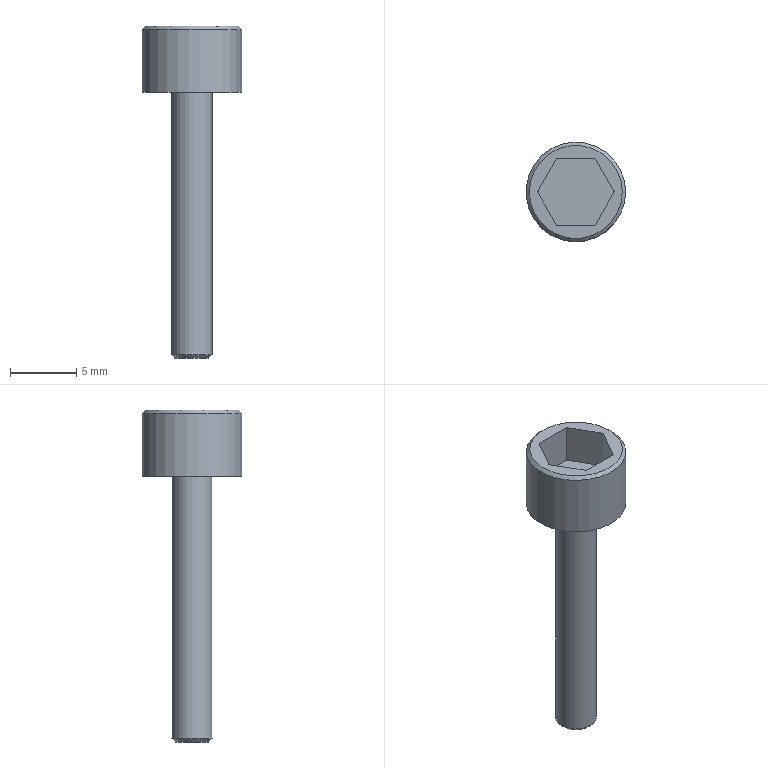Component | NX | SCREW | 1 solid | 14 faces | box 7.5 x 7.5 x 25 mm | volume 301 mm3 | plane 10 | cylinder 2 | cone 2 | commonest cylinder face diameters 3.045 x1 7.5 x1
STEP:
#1=CARTESIAN_POINT('',(0.,0.,0.));
#2=DIRECTION('',(0.,0.,1.));
#3=DIRECTION('',(1.,0.,0.));
#4=AXIS2_PLACEMENT_3D('',#1,#2,#3);
#5=CARTESIAN_POINT('',(23.5,-13.5,10.));
#6=VERTEX_POINT('',#5);
#7=CARTESIAN_POINT('',(20.,-13.5,10.));
#8=DIRECTION('',(0.,0.,1.));
#9=DIRECTION('',(1.,0.,0.));
#10=AXIS2_PLACEMENT_3D('',#7,#8,#9);
#11=CIRCLE('',#10,3.5);
#12=CARTESIAN_POINT('',(20.,-13.5,10.));
#13=DIRECTION('',(0.,0.,1.));
#14=DIRECTION('',(1.,0.,0.));
#15=AXIS2_PLACEMENT_3D('',#12,#13,#14);
#16=PLANE('',#15);
#17=CARTESIAN_POINT('',(0.,0.));
#18=DIRECTION('',(1.,0.));
#19=AXIS2_PLACEMENT_2D('',#17,#18);
#20=CIRCLE('',#19,3.5);
#21=(GEOMETRIC_REPRESENTATION_CONTEXT(2)PARAMETRIC_REPRESENTATION_CONTEXT()REPRESENTATION_CONTEXT('',''));
#22=DEFINITIONAL_REPRESENTATION('',(#20),#21);
#23=PCURVE('',#16,#22);
#24=CARTESIAN_POINT('',(20.,-13.5,10.));
#25=DIRECTION('',(0.,0.,-1.));
#26=DIRECTION('',(-1.,0.,0.));
#27=AXIS2_PLACEMENT_3D('',#24,#25,#26);
#28=CONICAL_SURFACE('',#27,3.5,0.7854);
#29=CARTESIAN_POINT('',(9.425,0.));
#30=DIRECTION('',(-1.,0.));
#31=VECTOR('',#30,1.);
#32=LINE('',#29,#31);
#33=(GEOMETRIC_REPRESENTATION_CONTEXT(2)PARAMETRIC_REPRESENTATION_CONTEXT()REPRESENTATION_CONTEXT('',''));
#34=DEFINITIONAL_REPRESENTATION('',(#32),#33);
#35=PCURVE('',#28,#34);
#36=SURFACE_CURVE('',#11,(#23,#35),.PCURVE_S1.);
#37=EDGE_CURVE('',#6,#6,#36,.T.);
#38=ORIENTED_EDGE('',*,*,#37,.T.);
#39=EDGE_LOOP('',(#38));
#40=FACE_BOUND('',#39,.T.);
#41=CARTESIAN_POINT('',(21.443,-11.,10.));
#42=VERTEX_POINT('',#41);
#43=CARTESIAN_POINT('',(22.887,-13.5,10.));
#44=VERTEX_POINT('',#43);
#45=CARTESIAN_POINT('',(21.443,-11.,10.));
#46=DIRECTION('',(0.5,-0.866,0.));
#47=VECTOR('',#46,1.);
#48=LINE('',#45,#47);
#49=CARTESIAN_POINT('',(1.443,2.5));
#50=DIRECTION('',(0.5,-0.866));
#51=VECTOR('',#50,1.);
#52=LINE('',#49,#51);
#53=(GEOMETRIC_REPRESENTATION_CONTEXT(2)PARAMETRIC_REPRESENTATION_CONTEXT()REPRESENTATION_CONTEXT('',''));
#54=DEFINITIONAL_REPRESENTATION('',(#52),#53);
#55=PCURVE('',#16,#54);
#56=CARTESIAN_POINT('',(21.443,-11.,7.));
#57=DIRECTION('',(-0.866,-0.5,0.));
#58=DIRECTION('',(0.5,-0.866,0.));
#59=AXIS2_PLACEMENT_3D('',#56,#57,#58);
#60=PLANE('',#59);
#61=CARTESIAN_POINT('',(0.,3.));
#62=DIRECTION('',(1.,0.));
#63=VECTOR('',#62,1.);
#64=LINE('',#61,#63);
#65=(GEOMETRIC_REPRESENTATION_CONTEXT(2)PARAMETRIC_REPRESENTATION_CONTEXT()REPRESENTATION_CONTEXT('',''));
#66=DEFINITIONAL_REPRESENTATION('',(#64),#65);
#67=PCURVE('',#60,#66);
#68=SURFACE_CURVE('',#48,(#55,#67),.PCURVE_S1.);
#69=EDGE_CURVE('',#42,#44,#68,.T.);
#70=ORIENTED_EDGE('',*,*,#69,.T.);
#71=CARTESIAN_POINT('',(21.443,-16.,10.));
#72=VERTEX_POINT('',#71);
#73=CARTESIAN_POINT('',(22.887,-13.5,10.));
#74=DIRECTION('',(-0.5,-0.866,0.));
#75=VECTOR('',#74,1.);
#76=LINE('',#73,#75);
#77=CARTESIAN_POINT('',(2.887,0.));
#78=DIRECTION('',(-0.5,-0.866));
#79=VECTOR('',#78,1.);
#80=LINE('',#77,#79);
#81=(GEOMETRIC_REPRESENTATION_CONTEXT(2)PARAMETRIC_REPRESENTATION_CONTEXT()REPRESENTATION_CONTEXT('',''));
#82=DEFINITIONAL_REPRESENTATION('',(#80),#81);
#83=PCURVE('',#16,#82);
#84=CARTESIAN_POINT('',(22.887,-13.5,7.));
#85=DIRECTION('',(-0.866,0.5,0.));
#86=DIRECTION('',(-0.5,-0.866,0.));
#87=AXIS2_PLACEMENT_3D('',#84,#85,#86);
#88=PLANE('',#87);
#89=CARTESIAN_POINT('',(0.,3.));
#90=DIRECTION('',(1.,0.));
#91=VECTOR('',#90,1.);
#92=LINE('',#89,#91);
#93=(GEOMETRIC_REPRESENTATION_CONTEXT(2)PARAMETRIC_REPRESENTATION_CONTEXT()REPRESENTATION_CONTEXT('',''));
#94=DEFINITIONAL_REPRESENTATION('',(#92),#93);
#95=PCURVE('',#88,#94);
#96=SURFACE_CURVE('',#76,(#83,#95),.PCURVE_S1.);
#97=EDGE_CURVE('',#44,#72,#96,.T.);
#98=ORIENTED_EDGE('',*,*,#97,.T.);
#99=CARTESIAN_POINT('',(18.557,-16.,10.));
#100=VERTEX_POINT('',#99);
#101=CARTESIAN_POINT('',(21.443,-16.,10.));
#102=DIRECTION('',(-1.,0.,0.));
#103=VECTOR('',#102,1.);
#104=LINE('',#101,#103);
#105=CARTESIAN_POINT('',(1.443,-2.5));
#106=DIRECTION('',(-1.,0.));
#107=VECTOR('',#106,1.);
#108=LINE('',#105,#107);
#109=(GEOMETRIC_REPRESENTATION_CONTEXT(2)PARAMETRIC_REPRESENTATION_CONTEXT()REPRESENTATION_CONTEXT('',''));
#110=DEFINITIONAL_REPRESENTATION('',(#108),#109);
#111=PCURVE('',#16,#110);
#112=CARTESIAN_POINT('',(21.443,-16.,7.));
#113=DIRECTION('',(0.,1.,0.));
#114=DIRECTION('',(-1.,0.,0.));
#115=AXIS2_PLACEMENT_3D('',#112,#113,#114);
#116=PLANE('',#115);
#117=CARTESIAN_POINT('',(0.,3.));
#118=DIRECTION('',(1.,0.));
#119=VECTOR('',#118,1.);
#120=LINE('',#117,#119);
#121=(GEOMETRIC_REPRESENTATION_CONTEXT(2)PARAMETRIC_REPRESENTATION_CONTEXT()REPRESENTATION_CONTEXT('',''));
#122=DEFINITIONAL_REPRESENTATION('',(#120),#121);
#123=PCURVE('',#116,#122);
#124=SURFACE_CURVE('',#104,(#111,#123),.PCURVE_S1.);
#125=EDGE_CURVE('',#72,#100,#124,.T.);
#126=ORIENTED_EDGE('',*,*,#125,.T.);
#127=CARTESIAN_POINT('',(17.113,-13.5,10.));
#128=VERTEX_POINT('',#127);
#129=CARTESIAN_POINT('',(18.557,-16.,10.));
#130=DIRECTION('',(-0.5,0.866,0.));
#131=VECTOR('',#130,1.);
#132=LINE('',#129,#131);
#133=CARTESIAN_POINT('',(-1.443,-2.5));
#134=DIRECTION('',(-0.5,0.866));
#135=VECTOR('',#134,1.);
#136=LINE('',#133,#135);
#137=(GEOMETRIC_REPRESENTATION_CONTEXT(2)PARAMETRIC_REPRESENTATION_CONTEXT()REPRESENTATION_CONTEXT('',''));
#138=DEFINITIONAL_REPRESENTATION('',(#136),#137);
#139=PCURVE('',#16,#138);
#140=CARTESIAN_POINT('',(18.557,-16.,7.));
#141=DIRECTION('',(0.866,0.5,0.));
#142=DIRECTION('',(-0.5,0.866,0.));
#143=AXIS2_PLACEMENT_3D('',#140,#141,#142);
#144=PLANE('',#143);
#145=CARTESIAN_POINT('',(0.,3.));
#146=DIRECTION('',(1.,0.));
#147=VECTOR('',#146,1.);
#148=LINE('',#145,#147);
#149=(GEOMETRIC_REPRESENTATION_CONTEXT(2)PARAMETRIC_REPRESENTATION_CONTEXT()REPRESENTATION_CONTEXT('',''));
#150=DEFINITIONAL_REPRESENTATION('',(#148),#149);
#151=PCURVE('',#144,#150);
#152=SURFACE_CURVE('',#132,(#139,#151),.PCURVE_S1.);
#153=EDGE_CURVE('',#100,#128,#152,.T.);
#154=ORIENTED_EDGE('',*,*,#153,.T.);
#155=CARTESIAN_POINT('',(18.557,-11.,10.));
#156=VERTEX_POINT('',#155);
#157=CARTESIAN_POINT('',(17.113,-13.5,10.));
#158=DIRECTION('',(0.5,0.866,0.));
#159=VECTOR('',#158,1.);
#160=LINE('',#157,#159);
#161=CARTESIAN_POINT('',(-2.887,0.));
#162=DIRECTION('',(0.5,0.866));
#163=VECTOR('',#162,1.);
#164=LINE('',#161,#163);
#165=(GEOMETRIC_REPRESENTATION_CONTEXT(2)PARAMETRIC_REPRESENTATION_CONTEXT()REPRESENTATION_CONTEXT('',''));
#166=DEFINITIONAL_REPRESENTATION('',(#164),#165);
#167=PCURVE('',#16,#166);
#168=CARTESIAN_POINT('',(17.113,-13.5,7.));
#169=DIRECTION('',(0.866,-0.5,0.));
#170=DIRECTION('',(0.5,0.866,0.));
#171=AXIS2_PLACEMENT_3D('',#168,#169,#170);
#172=PLANE('',#171);
#173=CARTESIAN_POINT('',(0.,3.));
#174=DIRECTION('',(1.,0.));
#175=VECTOR('',#174,1.);
#176=LINE('',#173,#175);
#177=(GEOMETRIC_REPRESENTATION_CONTEXT(2)PARAMETRIC_REPRESENTATION_CONTEXT()REPRESENTATION_CONTEXT('',''));
#178=DEFINITIONAL_REPRESENTATION('',(#176),#177);
#179=PCURVE('',#172,#178);
#180=SURFACE_CURVE('',#160,(#167,#179),.PCURVE_S1.);
#181=EDGE_CURVE('',#128,#156,#180,.T.);
#182=ORIENTED_EDGE('',*,*,#181,.T.);
#183=CARTESIAN_POINT('',(18.557,-11.,10.));
#184=DIRECTION('',(1.,0.,0.));
#185=VECTOR('',#184,1.);
#186=LINE('',#183,#185);
#187=CARTESIAN_POINT('',(-1.443,2.5));
#188=DIRECTION('',(1.,0.));
#189=VECTOR('',#188,1.);
#190=LINE('',#187,#189);
#191=(GEOMETRIC_REPRESENTATION_CONTEXT(2)PARAMETRIC_REPRESENTATION_CONTEXT()REPRESENTATION_CONTEXT('',''));
#192=DEFINITIONAL_REPRESENTATION('',(#190),#191);
#193=PCURVE('',#16,#192);
#194=CARTESIAN_POINT('',(18.557,-11.,7.));
#195=DIRECTION('',(0.,-1.,0.));
#196=DIRECTION('',(1.,0.,0.));
#197=AXIS2_PLACEMENT_3D('',#194,#195,#196);
#198=PLANE('',#197);
#199=CARTESIAN_POINT('',(0.,3.));
#200=DIRECTION('',(1.,0.));
#201=VECTOR('',#200,1.);
#202=LINE('',#199,#201);
#203=(GEOMETRIC_REPRESENTATION_CONTEXT(2)PARAMETRIC_REPRESENTATION_CONTEXT()REPRESENTATION_CONTEXT('',''));
#204=DEFINITIONAL_REPRESENTATION('',(#202),#203);
#205=PCURVE('',#198,#204);
#206=SURFACE_CURVE('',#186,(#193,#205),.PCURVE_S1.);
#207=EDGE_CURVE('',#156,#42,#206,.T.);
#208=ORIENTED_EDGE('',*,*,#207,.T.);
#209=EDGE_LOOP('',(#70,#98,#126,#154,#182,#208));
#210=FACE_BOUND('',#209,.T.);
#211=ADVANCED_FACE('',(#40,#210),#16,.T.);
#212=CARTESIAN_POINT('',(18.727,-13.5,-15.));
#213=VERTEX_POINT('',#212);
#214=CARTESIAN_POINT('',(20.,-13.5,-15.));
#215=DIRECTION('',(0.,0.,-1.));
#216=DIRECTION('',(-1.,0.,0.));
#217=AXIS2_PLACEMENT_3D('',#214,#215,#216);
#218=CIRCLE('',#217,1.273);
#219=CARTESIAN_POINT('',(20.,-13.5,-15.));
#220=DIRECTION('',(0.,0.,-1.));
#221=DIRECTION('',(-1.,0.,0.));
#222=AXIS2_PLACEMENT_3D('',#219,#220,#221);
#223=PLANE('',#222);
#224=CARTESIAN_POINT('',(0.,0.));
#225=DIRECTION('',(1.,0.));
#226=AXIS2_PLACEMENT_2D('',#224,#225);
#227=CIRCLE('',#226,1.273);
#228=(GEOMETRIC_REPRESENTATION_CONTEXT(2)PARAMETRIC_REPRESENTATION_CONTEXT()REPRESENTATION_CONTEXT('',''));
#229=DEFINITIONAL_REPRESENTATION('',(#227),#228);
#230=PCURVE('',#223,#229);
#231=CARTESIAN_POINT('',(20.,-13.5,-14.75));
#232=DIRECTION('',(0.,0.,1.));
#233=DIRECTION('',(1.,0.,0.));
#234=AXIS2_PLACEMENT_3D('',#231,#232,#233);
#235=CONICAL_SURFACE('',#234,1.523,0.7854);
#236=CARTESIAN_POINT('',(9.425,-0.25));
#237=DIRECTION('',(-1.,0.));
#238=VECTOR('',#237,1.);
#239=LINE('',#236,#238);
#240=(GEOMETRIC_REPRESENTATION_CONTEXT(2)PARAMETRIC_REPRESENTATION_CONTEXT()REPRESENTATION_CONTEXT('',''));
#241=DEFINITIONAL_REPRESENTATION('',(#239),#240);
#242=PCURVE('',#235,#241);
#243=SURFACE_CURVE('',#218,(#230,#242),.PCURVE_S1.);
#244=EDGE_CURVE('',#213,#213,#243,.T.);
#245=ORIENTED_EDGE('',*,*,#244,.T.);
#246=EDGE_LOOP('',(#245));
#247=FACE_BOUND('',#246,.T.);
#248=ADVANCED_FACE('',(#247),#223,.T.);
#249=CARTESIAN_POINT('',(18.477,-13.5,-14.75));
#250=VERTEX_POINT('',#249);
#251=CARTESIAN_POINT('',(21.523,-13.5,-14.75));
#252=VERTEX_POINT('',#251);
#253=CARTESIAN_POINT('',(20.,-13.5,-14.75));
#254=DIRECTION('',(0.,0.,1.));
#255=DIRECTION('',(-1.,0.,0.));
#256=AXIS2_PLACEMENT_3D('',#253,#254,#255);
#257=CIRCLE('',#256,1.523);
#258=CARTESIAN_POINT('',(20.,-13.5,-15.));
#259=DIRECTION('',(0.,0.,1.));
#260=DIRECTION('',(1.,0.,0.));
#261=AXIS2_PLACEMENT_3D('',#258,#259,#260);
#262=CYLINDRICAL_SURFACE('',#261,1.523);
#263=CARTESIAN_POINT('',(3.142,0.25));
#264=DIRECTION('',(1.,0.));
#265=VECTOR('',#264,1.);
#266=LINE('',#263,#265);
#267=(GEOMETRIC_REPRESENTATION_CONTEXT(2)PARAMETRIC_REPRESENTATION_CONTEXT()REPRESENTATION_CONTEXT('',''));
#268=DEFINITIONAL_REPRESENTATION('',(#266),#267);
#269=PCURVE('',#262,#268);
#270=CARTESIAN_POINT('',(3.142,-0.));
#271=DIRECTION('',(1.,0.));
#272=VECTOR('',#271,1.);
#273=LINE('',#270,#272);
#274=(GEOMETRIC_REPRESENTATION_CONTEXT(2)PARAMETRIC_REPRESENTATION_CONTEXT()REPRESENTATION_CONTEXT('',''));
#275=DEFINITIONAL_REPRESENTATION('',(#273),#274);
#276=PCURVE('',#235,#275);
#277=SURFACE_CURVE('',#257,(#269,#276),.PCURVE_S1.);
#278=EDGE_CURVE('',#250,#252,#277,.T.);
#279=ORIENTED_EDGE('',*,*,#278,.T.);
#280=CARTESIAN_POINT('',(21.523,-13.5,5.));
#281=VERTEX_POINT('',#280);
#282=CARTESIAN_POINT('',(21.523,-13.5,-14.75));
#283=CARTESIAN_POINT('',(21.523,-13.5,5.));
#284=B_SPLINE_CURVE_WITH_KNOTS('',1,(#282,#283),.UNSPECIFIED.,.F.,.F.,(2,2),(0.25,20.),.PIECEWISE_BEZIER_KNOTS.);
#285=CARTESIAN_POINT('',(6.283,0.));
#286=DIRECTION('',(0.,1.));
#287=VECTOR('',#286,1.);
#288=LINE('',#285,#287);
#289=(GEOMETRIC_REPRESENTATION_CONTEXT(2)PARAMETRIC_REPRESENTATION_CONTEXT()REPRESENTATION_CONTEXT('',''));
#290=DEFINITIONAL_REPRESENTATION('',(#288),#289);
#291=PCURVE('',#262,#290);
#292=CARTESIAN_POINT('',(0.,0.));
#293=DIRECTION('',(0.,1.));
#294=VECTOR('',#293,1.);
#295=LINE('',#292,#294);
#296=(GEOMETRIC_REPRESENTATION_CONTEXT(2)PARAMETRIC_REPRESENTATION_CONTEXT()REPRESENTATION_CONTEXT('',''));
#297=DEFINITIONAL_REPRESENTATION('',(#295),#296);
#298=PCURVE('',#262,#297);
#299=SEAM_CURVE('',#284,(#291,#298),.PCURVE_S1.);
#300=EDGE_CURVE('',#252,#281,#299,.T.);
#301=ORIENTED_EDGE('',*,*,#300,.T.);
#302=CARTESIAN_POINT('',(20.,-13.5,5.));
#303=DIRECTION('',(0.,0.,-1.));
#304=DIRECTION('',(1.,0.,0.));
#305=AXIS2_PLACEMENT_3D('',#302,#303,#304);
#306=CIRCLE('',#305,1.523);
#307=CARTESIAN_POINT('',(6.283,20.));
#308=DIRECTION('',(-1.,0.));
#309=VECTOR('',#308,1.);
#310=LINE('',#307,#309);
#311=(GEOMETRIC_REPRESENTATION_CONTEXT(2)PARAMETRIC_REPRESENTATION_CONTEXT()REPRESENTATION_CONTEXT('',''));
#312=DEFINITIONAL_REPRESENTATION('',(#310),#311);
#313=PCURVE('',#262,#312);
#314=CARTESIAN_POINT('',(20.,-13.5,5.));
#315=DIRECTION('',(0.,0.,-1.));
#316=DIRECTION('',(-1.,0.,0.));
#317=AXIS2_PLACEMENT_3D('',#314,#315,#316);
#318=PLANE('',#317);
#319=CARTESIAN_POINT('',(0.,0.));
#320=DIRECTION('',(-1.,0.));
#321=AXIS2_PLACEMENT_2D('',#319,#320);
#322=CIRCLE('',#321,1.523);
#323=(GEOMETRIC_REPRESENTATION_CONTEXT(2)PARAMETRIC_REPRESENTATION_CONTEXT()REPRESENTATION_CONTEXT('',''));
#324=DEFINITIONAL_REPRESENTATION('',(#322),#323);
#325=PCURVE('',#318,#324);
#326=SURFACE_CURVE('',#306,(#313,#325),.PCURVE_S1.);
#327=EDGE_CURVE('',#281,#281,#326,.T.);
#328=ORIENTED_EDGE('',*,*,#327,.T.);
#329=ORIENTED_EDGE('',*,*,#300,.F.);
#330=CARTESIAN_POINT('',(20.,-13.5,-14.75));
#331=DIRECTION('',(0.,0.,1.));
#332=DIRECTION('',(-1.,0.,0.));
#333=AXIS2_PLACEMENT_3D('',#330,#331,#332);
#334=CIRCLE('',#333,1.523);
#335=CARTESIAN_POINT('',(-3.142,0.25));
#336=DIRECTION('',(1.,0.));
#337=VECTOR('',#336,1.);
#338=LINE('',#335,#337);
#339=(GEOMETRIC_REPRESENTATION_CONTEXT(2)PARAMETRIC_REPRESENTATION_CONTEXT()REPRESENTATION_CONTEXT('',''));
#340=DEFINITIONAL_REPRESENTATION('',(#338),#339);
#341=PCURVE('',#262,#340);
#342=CARTESIAN_POINT('',(3.142,-0.));
#343=DIRECTION('',(1.,0.));
#344=VECTOR('',#343,1.);
#345=LINE('',#342,#344);
#346=(GEOMETRIC_REPRESENTATION_CONTEXT(2)PARAMETRIC_REPRESENTATION_CONTEXT()REPRESENTATION_CONTEXT('',''));
#347=DEFINITIONAL_REPRESENTATION('',(#345),#346);
#348=PCURVE('',#235,#347);
#349=SURFACE_CURVE('',#334,(#341,#348),.PCURVE_S1.);
#350=EDGE_CURVE('',#252,#250,#349,.T.);
#351=ORIENTED_EDGE('',*,*,#350,.T.);
#352=EDGE_LOOP('',(#279,#301,#328,#329,#351));
#353=FACE_BOUND('',#352,.T.);
#354=ADVANCED_FACE('',(#353),#262,.T.);
#355=ORIENTED_EDGE('',*,*,#327,.F.);
#356=EDGE_LOOP('',(#355));
#357=FACE_BOUND('',#356,.T.);
#358=CARTESIAN_POINT('',(23.75,-13.5,5.));
#359=VERTEX_POINT('',#358);
#360=CARTESIAN_POINT('',(20.,-13.5,5.));
#361=DIRECTION('',(0.,0.,1.));
#362=DIRECTION('',(1.,0.,0.));
#363=AXIS2_PLACEMENT_3D('',#360,#361,#362);
#364=CIRCLE('',#363,3.75);
#365=CARTESIAN_POINT('',(-3.75,0.));
#366=CARTESIAN_POINT('',(-3.75,6.495));
#367=CARTESIAN_POINT('',(1.875,3.248));
#368=CARTESIAN_POINT('',(7.5,0.));
#369=CARTESIAN_POINT('',(1.875,-3.248));
#370=CARTESIAN_POINT('',(-3.75,-6.495));
#371=CARTESIAN_POINT('',(-3.75,0.));
#372=(BOUNDED_CURVE()B_SPLINE_CURVE(2,(#365,#366,#367,#368,#369,#370,#371),.UNSPECIFIED.,.T.,.F.)B_SPLINE_CURVE_WITH_KNOTS((1,2,2,2,2,1),(-2.094,0.,2.094,4.189,6.283,8.378),.UNSPECIFIED.)CURVE()GEOMETRIC_REPRESENTATION_ITEM()RATIONAL_B_SPLINE_CURVE((1.,0.5,1.,0.5,1.,0.5,1.))REPRESENTATION_ITEM(''));
#373=(GEOMETRIC_REPRESENTATION_CONTEXT(2)PARAMETRIC_REPRESENTATION_CONTEXT()REPRESENTATION_CONTEXT('',''));
#374=DEFINITIONAL_REPRESENTATION('',(#372),#373);
#375=PCURVE('',#318,#374);
#376=CARTESIAN_POINT('',(20.,-13.5,5.));
#377=DIRECTION('',(0.,0.,1.));
#378=DIRECTION('',(1.,0.,0.));
#379=AXIS2_PLACEMENT_3D('',#376,#377,#378);
#380=CYLINDRICAL_SURFACE('',#379,3.75);
#381=CARTESIAN_POINT('',(0.,0.));
#382=DIRECTION('',(1.,0.));
#383=VECTOR('',#382,1.);
#384=LINE('',#381,#383);
#385=(GEOMETRIC_REPRESENTATION_CONTEXT(2)PARAMETRIC_REPRESENTATION_CONTEXT()REPRESENTATION_CONTEXT('',''));
#386=DEFINITIONAL_REPRESENTATION('',(#384),#385);
#387=PCURVE('',#380,#386);
#388=SURFACE_CURVE('',#364,(#375,#387),.PCURVE_S1.);
#389=EDGE_CURVE('',#359,#359,#388,.T.);
#390=ORIENTED_EDGE('',*,*,#389,.F.);
#391=EDGE_LOOP('',(#390));
#392=FACE_BOUND('',#391,.T.);
#393=ADVANCED_FACE('',(#357,#392),#318,.T.);
#394=CARTESIAN_POINT('',(23.75,-13.5,9.75));
#395=VERTEX_POINT('',#394);
#396=CARTESIAN_POINT('',(20.,-13.5,9.75));
#397=DIRECTION('',(0.,0.,-1.));
#398=DIRECTION('',(1.,0.,0.));
#399=AXIS2_PLACEMENT_3D('',#396,#397,#398);
#400=CIRCLE('',#399,3.75);
#401=CARTESIAN_POINT('',(6.283,4.75));
#402=DIRECTION('',(-1.,0.));
#403=VECTOR('',#402,1.);
#404=LINE('',#401,#403);
#405=(GEOMETRIC_REPRESENTATION_CONTEXT(2)PARAMETRIC_REPRESENTATION_CONTEXT()REPRESENTATION_CONTEXT('',''));
#406=DEFINITIONAL_REPRESENTATION('',(#404),#405);
#407=PCURVE('',#380,#406);
#408=CARTESIAN_POINT('',(3.142,0.25));
#409=DIRECTION('',(1.,0.));
#410=VECTOR('',#409,1.);
#411=LINE('',#408,#410);
#412=(GEOMETRIC_REPRESENTATION_CONTEXT(2)PARAMETRIC_REPRESENTATION_CONTEXT()REPRESENTATION_CONTEXT('',''));
#413=DEFINITIONAL_REPRESENTATION('',(#411),#412);
#414=PCURVE('',#28,#413);
#415=SURFACE_CURVE('',#400,(#407,#414),.PCURVE_S1.);
#416=EDGE_CURVE('',#395,#395,#415,.T.);
#417=ORIENTED_EDGE('',*,*,#416,.T.);
#418=CARTESIAN_POINT('',(23.75,-13.5,5.));
#419=CARTESIAN_POINT('',(23.75,-13.5,9.75));
#420=B_SPLINE_CURVE_WITH_KNOTS('',1,(#418,#419),.UNSPECIFIED.,.F.,.F.,(2,2),(0.,4.75),.PIECEWISE_BEZIER_KNOTS.);
#421=CARTESIAN_POINT('',(0.,0.));
#422=DIRECTION('',(0.,1.));
#423=VECTOR('',#422,1.);
#424=LINE('',#421,#423);
#425=(GEOMETRIC_REPRESENTATION_CONTEXT(2)PARAMETRIC_REPRESENTATION_CONTEXT()REPRESENTATION_CONTEXT('',''));
#426=DEFINITIONAL_REPRESENTATION('',(#424),#425);
#427=PCURVE('',#380,#426);
#428=CARTESIAN_POINT('',(6.283,0.));
#429=DIRECTION('',(0.,1.));
#430=VECTOR('',#429,1.);
#431=LINE('',#428,#430);
#432=(GEOMETRIC_REPRESENTATION_CONTEXT(2)PARAMETRIC_REPRESENTATION_CONTEXT()REPRESENTATION_CONTEXT('',''));
#433=DEFINITIONAL_REPRESENTATION('',(#431),#432);
#434=PCURVE('',#380,#433);
#435=SEAM_CURVE('',#420,(#427,#434),.PCURVE_S1.);
#436=EDGE_CURVE('',#359,#395,#435,.T.);
#437=ORIENTED_EDGE('',*,*,#436,.F.);
#438=ORIENTED_EDGE('',*,*,#389,.T.);
#439=ORIENTED_EDGE('',*,*,#436,.T.);
#440=EDGE_LOOP('',(#417,#437,#438,#439));
#441=FACE_BOUND('',#440,.T.);
#442=ADVANCED_FACE('',(#441),#380,.T.);
#443=ORIENTED_EDGE('',*,*,#244,.F.);
#444=CARTESIAN_POINT('',(18.727,-13.5,-15.));
#445=CARTESIAN_POINT('',(18.477,-13.5,-14.75));
#446=B_SPLINE_CURVE_WITH_KNOTS('',1,(#444,#445),.UNSPECIFIED.,.F.,.F.,(2,2),(-0.3536,-0.),.PIECEWISE_BEZIER_KNOTS.);
#447=CARTESIAN_POINT('',(9.425,0.));
#448=DIRECTION('',(0.,1.));
#449=VECTOR('',#448,1.);
#450=LINE('',#447,#449);
#451=(GEOMETRIC_REPRESENTATION_CONTEXT(2)PARAMETRIC_REPRESENTATION_CONTEXT()REPRESENTATION_CONTEXT('',''));
#452=DEFINITIONAL_REPRESENTATION('',(#450),#451);
#453=PCURVE('',#235,#452);
#454=CARTESIAN_POINT('',(3.142,0.));
#455=DIRECTION('',(0.,1.));
#456=VECTOR('',#455,1.);
#457=LINE('',#454,#456);
#458=(GEOMETRIC_REPRESENTATION_CONTEXT(2)PARAMETRIC_REPRESENTATION_CONTEXT()REPRESENTATION_CONTEXT('',''));
#459=DEFINITIONAL_REPRESENTATION('',(#457),#458);
#460=PCURVE('',#235,#459);
#461=SEAM_CURVE('',#446,(#453,#460),.PCURVE_S1.);
#462=EDGE_CURVE('',#213,#250,#461,.T.);
#463=ORIENTED_EDGE('',*,*,#462,.T.);
#464=ORIENTED_EDGE('',*,*,#350,.F.);
#465=ORIENTED_EDGE('',*,*,#278,.F.);
#466=ORIENTED_EDGE('',*,*,#462,.F.);
#467=EDGE_LOOP('',(#443,#463,#464,#465,#466));
#468=FACE_BOUND('',#467,.T.);
#469=ADVANCED_FACE('',(#468),#235,.T.);
#470=ORIENTED_EDGE('',*,*,#97,.F.);
#471=CARTESIAN_POINT('',(22.887,-13.5,7.));
#472=VERTEX_POINT('',#471);
#473=CARTESIAN_POINT('',(22.887,-13.5,7.));
#474=DIRECTION('',(0.,0.,-1.));
#475=VECTOR('',#474,1.);
#476=LINE('',#473,#475);
#477=CARTESIAN_POINT('',(0.,0.));
#478=DIRECTION('',(0.,-1.));
#479=VECTOR('',#478,1.);
#480=LINE('',#477,#479);
#481=(GEOMETRIC_REPRESENTATION_CONTEXT(2)PARAMETRIC_REPRESENTATION_CONTEXT()REPRESENTATION_CONTEXT('',''));
#482=DEFINITIONAL_REPRESENTATION('',(#480),#481);
#483=PCURVE('',#88,#482);
#484=CARTESIAN_POINT('',(2.887,0.));
#485=DIRECTION('',(0.,-1.));
#486=VECTOR('',#485,1.);
#487=LINE('',#484,#486);
#488=(GEOMETRIC_REPRESENTATION_CONTEXT(2)PARAMETRIC_REPRESENTATION_CONTEXT()REPRESENTATION_CONTEXT('',''));
#489=DEFINITIONAL_REPRESENTATION('',(#487),#488);
#490=PCURVE('',#60,#489);
#491=SURFACE_CURVE('',#476,(#483,#490),.PCURVE_S1.);
#492=EDGE_CURVE('',#44,#472,#491,.T.);
#493=ORIENTED_EDGE('',*,*,#492,.T.);
#494=CARTESIAN_POINT('',(21.443,-16.,7.));
#495=VERTEX_POINT('',#494);
#496=CARTESIAN_POINT('',(22.887,-13.5,7.));
#497=DIRECTION('',(0.5,0.866,0.));
#498=VECTOR('',#497,1.);
#499=LINE('',#496,#498);
#500=CARTESIAN_POINT('',(0.,0.));
#501=DIRECTION('',(-1.,0.));
#502=VECTOR('',#501,1.);
#503=LINE('',#500,#502);
#504=(GEOMETRIC_REPRESENTATION_CONTEXT(2)PARAMETRIC_REPRESENTATION_CONTEXT()REPRESENTATION_CONTEXT('',''));
#505=DEFINITIONAL_REPRESENTATION('',(#503),#504);
#506=PCURVE('',#88,#505);
#507=CARTESIAN_POINT('',(20.,-13.5,7.));
#508=DIRECTION('',(0.,0.,-1.));
#509=DIRECTION('',(-1.,0.,0.));
#510=AXIS2_PLACEMENT_3D('',#507,#508,#509);
#511=PLANE('',#510);
#512=CARTESIAN_POINT('',(-2.887,0.));
#513=DIRECTION('',(-0.5,0.866));
#514=VECTOR('',#513,1.);
#515=LINE('',#512,#514);
#516=(GEOMETRIC_REPRESENTATION_CONTEXT(2)PARAMETRIC_REPRESENTATION_CONTEXT()REPRESENTATION_CONTEXT('',''));
#517=DEFINITIONAL_REPRESENTATION('',(#515),#516);
#518=PCURVE('',#511,#517);
#519=SURFACE_CURVE('',#499,(#506,#518),.PCURVE_S1.);
#520=EDGE_CURVE('',#495,#472,#519,.T.);
#521=ORIENTED_EDGE('',*,*,#520,.F.);
#522=CARTESIAN_POINT('',(21.443,-16.,7.));
#523=DIRECTION('',(0.,0.,-1.));
#524=VECTOR('',#523,1.);
#525=LINE('',#522,#524);
#526=CARTESIAN_POINT('',(2.887,0.));
#527=DIRECTION('',(0.,-1.));
#528=VECTOR('',#527,1.);
#529=LINE('',#526,#528);
#530=(GEOMETRIC_REPRESENTATION_CONTEXT(2)PARAMETRIC_REPRESENTATION_CONTEXT()REPRESENTATION_CONTEXT('',''));
#531=DEFINITIONAL_REPRESENTATION('',(#529),#530);
#532=PCURVE('',#88,#531);
#533=CARTESIAN_POINT('',(0.,0.));
#534=DIRECTION('',(0.,-1.));
#535=VECTOR('',#534,1.);
#536=LINE('',#533,#535);
#537=(GEOMETRIC_REPRESENTATION_CONTEXT(2)PARAMETRIC_REPRESENTATION_CONTEXT()REPRESENTATION_CONTEXT('',''));
#538=DEFINITIONAL_REPRESENTATION('',(#536),#537);
#539=PCURVE('',#116,#538);
#540=SURFACE_CURVE('',#525,(#532,#539),.PCURVE_S1.);
#541=EDGE_CURVE('',#72,#495,#540,.T.);
#542=ORIENTED_EDGE('',*,*,#541,.F.);
#543=EDGE_LOOP('',(#470,#493,#521,#542));
#544=FACE_BOUND('',#543,.T.);
#545=ADVANCED_FACE('',(#544),#88,.T.);
#546=ORIENTED_EDGE('',*,*,#125,.F.);
#547=ORIENTED_EDGE('',*,*,#541,.T.);
#548=CARTESIAN_POINT('',(18.557,-16.,7.));
#549=VERTEX_POINT('',#548);
#550=CARTESIAN_POINT('',(21.443,-16.,7.));
#551=DIRECTION('',(1.,-0.,0.));
#552=VECTOR('',#551,1.);
#553=LINE('',#550,#552);
#554=CARTESIAN_POINT('',(0.,0.));
#555=DIRECTION('',(-1.,0.));
#556=VECTOR('',#555,1.);
#557=LINE('',#554,#556);
#558=(GEOMETRIC_REPRESENTATION_CONTEXT(2)PARAMETRIC_REPRESENTATION_CONTEXT()REPRESENTATION_CONTEXT('',''));
#559=DEFINITIONAL_REPRESENTATION('',(#557),#558);
#560=PCURVE('',#116,#559);
#561=CARTESIAN_POINT('',(-1.443,-2.5));
#562=DIRECTION('',(-1.,-0.));
#563=VECTOR('',#562,1.);
#564=LINE('',#561,#563);
#565=(GEOMETRIC_REPRESENTATION_CONTEXT(2)PARAMETRIC_REPRESENTATION_CONTEXT()REPRESENTATION_CONTEXT('',''));
#566=DEFINITIONAL_REPRESENTATION('',(#564),#565);
#567=PCURVE('',#511,#566);
#568=SURFACE_CURVE('',#553,(#560,#567),.PCURVE_S1.);
#569=EDGE_CURVE('',#549,#495,#568,.T.);
#570=ORIENTED_EDGE('',*,*,#569,.F.);
#571=CARTESIAN_POINT('',(18.557,-16.,7.));
#572=DIRECTION('',(0.,0.,-1.));
#573=VECTOR('',#572,1.);
#574=LINE('',#571,#573);
#575=CARTESIAN_POINT('',(2.887,0.));
#576=DIRECTION('',(0.,-1.));
#577=VECTOR('',#576,1.);
#578=LINE('',#575,#577);
#579=(GEOMETRIC_REPRESENTATION_CONTEXT(2)PARAMETRIC_REPRESENTATION_CONTEXT()REPRESENTATION_CONTEXT('',''));
#580=DEFINITIONAL_REPRESENTATION('',(#578),#579);
#581=PCURVE('',#116,#580);
#582=CARTESIAN_POINT('',(0.,0.));
#583=DIRECTION('',(0.,-1.));
#584=VECTOR('',#583,1.);
#585=LINE('',#582,#584);
#586=(GEOMETRIC_REPRESENTATION_CONTEXT(2)PARAMETRIC_REPRESENTATION_CONTEXT()REPRESENTATION_CONTEXT('',''));
#587=DEFINITIONAL_REPRESENTATION('',(#585),#586);
#588=PCURVE('',#144,#587);
#589=SURFACE_CURVE('',#574,(#581,#588),.PCURVE_S1.);
#590=EDGE_CURVE('',#100,#549,#589,.T.);
#591=ORIENTED_EDGE('',*,*,#590,.F.);
#592=EDGE_LOOP('',(#546,#547,#570,#591));
#593=FACE_BOUND('',#592,.T.);
#594=ADVANCED_FACE('',(#593),#116,.T.);
#595=ORIENTED_EDGE('',*,*,#153,.F.);
#596=ORIENTED_EDGE('',*,*,#590,.T.);
#597=CARTESIAN_POINT('',(17.113,-13.5,7.));
#598=VERTEX_POINT('',#597);
#599=CARTESIAN_POINT('',(18.557,-16.,7.));
#600=DIRECTION('',(0.5,-0.866,0.));
#601=VECTOR('',#600,1.);
#602=LINE('',#599,#601);
#603=CARTESIAN_POINT('',(0.,0.));
#604=DIRECTION('',(-1.,0.));
#605=VECTOR('',#604,1.);
#606=LINE('',#603,#605);
#607=(GEOMETRIC_REPRESENTATION_CONTEXT(2)PARAMETRIC_REPRESENTATION_CONTEXT()REPRESENTATION_CONTEXT('',''));
#608=DEFINITIONAL_REPRESENTATION('',(#606),#607);
#609=PCURVE('',#144,#608);
#610=CARTESIAN_POINT('',(1.443,-2.5));
#611=DIRECTION('',(-0.5,-0.866));
#612=VECTOR('',#611,1.);
#613=LINE('',#610,#612);
#614=(GEOMETRIC_REPRESENTATION_CONTEXT(2)PARAMETRIC_REPRESENTATION_CONTEXT()REPRESENTATION_CONTEXT('',''));
#615=DEFINITIONAL_REPRESENTATION('',(#613),#614);
#616=PCURVE('',#511,#615);
#617=SURFACE_CURVE('',#602,(#609,#616),.PCURVE_S1.);
#618=EDGE_CURVE('',#598,#549,#617,.T.);
#619=ORIENTED_EDGE('',*,*,#618,.F.);
#620=CARTESIAN_POINT('',(17.113,-13.5,7.));
#621=DIRECTION('',(0.,0.,-1.));
#622=VECTOR('',#621,1.);
#623=LINE('',#620,#622);
#624=CARTESIAN_POINT('',(2.887,0.));
#625=DIRECTION('',(0.,-1.));
#626=VECTOR('',#625,1.);
#627=LINE('',#624,#626);
#628=(GEOMETRIC_REPRESENTATION_CONTEXT(2)PARAMETRIC_REPRESENTATION_CONTEXT()REPRESENTATION_CONTEXT('',''));
#629=DEFINITIONAL_REPRESENTATION('',(#627),#628);
#630=PCURVE('',#144,#629);
#631=CARTESIAN_POINT('',(0.,0.));
#632=DIRECTION('',(0.,-1.));
#633=VECTOR('',#632,1.);
#634=LINE('',#631,#633);
#635=(GEOMETRIC_REPRESENTATION_CONTEXT(2)PARAMETRIC_REPRESENTATION_CONTEXT()REPRESENTATION_CONTEXT('',''));
#636=DEFINITIONAL_REPRESENTATION('',(#634),#635);
#637=PCURVE('',#172,#636);
#638=SURFACE_CURVE('',#623,(#630,#637),.PCURVE_S1.);
#639=EDGE_CURVE('',#128,#598,#638,.T.);
#640=ORIENTED_EDGE('',*,*,#639,.F.);
#641=EDGE_LOOP('',(#595,#596,#619,#640));
#642=FACE_BOUND('',#641,.T.);
#643=ADVANCED_FACE('',(#642),#144,.T.);
#644=ORIENTED_EDGE('',*,*,#181,.F.);
#645=ORIENTED_EDGE('',*,*,#639,.T.);
#646=CARTESIAN_POINT('',(18.557,-11.,7.));
#647=VERTEX_POINT('',#646);
#648=CARTESIAN_POINT('',(17.113,-13.5,7.));
#649=DIRECTION('',(-0.5,-0.866,0.));
#650=VECTOR('',#649,1.);
#651=LINE('',#648,#650);
#652=CARTESIAN_POINT('',(0.,0.));
#653=DIRECTION('',(-1.,0.));
#654=VECTOR('',#653,1.);
#655=LINE('',#652,#654);
#656=(GEOMETRIC_REPRESENTATION_CONTEXT(2)PARAMETRIC_REPRESENTATION_CONTEXT()REPRESENTATION_CONTEXT('',''));
#657=DEFINITIONAL_REPRESENTATION('',(#655),#656);
#658=PCURVE('',#172,#657);
#659=CARTESIAN_POINT('',(2.887,0.));
#660=DIRECTION('',(0.5,-0.866));
#661=VECTOR('',#660,1.);
#662=LINE('',#659,#661);
#663=(GEOMETRIC_REPRESENTATION_CONTEXT(2)PARAMETRIC_REPRESENTATION_CONTEXT()REPRESENTATION_CONTEXT('',''));
#664=DEFINITIONAL_REPRESENTATION('',(#662),#663);
#665=PCURVE('',#511,#664);
#666=SURFACE_CURVE('',#651,(#658,#665),.PCURVE_S1.);
#667=EDGE_CURVE('',#647,#598,#666,.T.);
#668=ORIENTED_EDGE('',*,*,#667,.F.);
#669=CARTESIAN_POINT('',(18.557,-11.,7.));
#670=DIRECTION('',(0.,0.,-1.));
#671=VECTOR('',#670,1.);
#672=LINE('',#669,#671);
#673=CARTESIAN_POINT('',(2.887,0.));
#674=DIRECTION('',(0.,-1.));
#675=VECTOR('',#674,1.);
#676=LINE('',#673,#675);
#677=(GEOMETRIC_REPRESENTATION_CONTEXT(2)PARAMETRIC_REPRESENTATION_CONTEXT()REPRESENTATION_CONTEXT('',''));
#678=DEFINITIONAL_REPRESENTATION('',(#676),#677);
#679=PCURVE('',#172,#678);
#680=CARTESIAN_POINT('',(0.,0.));
#681=DIRECTION('',(0.,-1.));
#682=VECTOR('',#681,1.);
#683=LINE('',#680,#682);
#684=(GEOMETRIC_REPRESENTATION_CONTEXT(2)PARAMETRIC_REPRESENTATION_CONTEXT()REPRESENTATION_CONTEXT('',''));
#685=DEFINITIONAL_REPRESENTATION('',(#683),#684);
#686=PCURVE('',#198,#685);
#687=SURFACE_CURVE('',#672,(#679,#686),.PCURVE_S1.);
#688=EDGE_CURVE('',#156,#647,#687,.T.);
#689=ORIENTED_EDGE('',*,*,#688,.F.);
#690=EDGE_LOOP('',(#644,#645,#668,#689));
#691=FACE_BOUND('',#690,.T.);
#692=ADVANCED_FACE('',(#691),#172,.T.);
#693=ORIENTED_EDGE('',*,*,#207,.F.);
#694=ORIENTED_EDGE('',*,*,#688,.T.);
#695=CARTESIAN_POINT('',(21.443,-11.,7.));
#696=VERTEX_POINT('',#695);
#697=CARTESIAN_POINT('',(18.557,-11.,7.));
#698=DIRECTION('',(-1.,-0.,0.));
#699=VECTOR('',#698,1.);
#700=LINE('',#697,#699);
#701=CARTESIAN_POINT('',(0.,0.));
#702=DIRECTION('',(-1.,0.));
#703=VECTOR('',#702,1.);
#704=LINE('',#701,#703);
#705=(GEOMETRIC_REPRESENTATION_CONTEXT(2)PARAMETRIC_REPRESENTATION_CONTEXT()REPRESENTATION_CONTEXT('',''));
#706=DEFINITIONAL_REPRESENTATION('',(#704),#705);
#707=PCURVE('',#198,#706);
#708=CARTESIAN_POINT('',(1.443,2.5));
#709=DIRECTION('',(1.,-0.));
#710=VECTOR('',#709,1.);
#711=LINE('',#708,#710);
#712=(GEOMETRIC_REPRESENTATION_CONTEXT(2)PARAMETRIC_REPRESENTATION_CONTEXT()REPRESENTATION_CONTEXT('',''));
#713=DEFINITIONAL_REPRESENTATION('',(#711),#712);
#714=PCURVE('',#511,#713);
#715=SURFACE_CURVE('',#700,(#707,#714),.PCURVE_S1.);
#716=EDGE_CURVE('',#696,#647,#715,.T.);
#717=ORIENTED_EDGE('',*,*,#716,.F.);
#718=CARTESIAN_POINT('',(21.443,-11.,7.));
#719=DIRECTION('',(0.,0.,-1.));
#720=VECTOR('',#719,1.);
#721=LINE('',#718,#720);
#722=CARTESIAN_POINT('',(2.887,0.));
#723=DIRECTION('',(0.,-1.));
#724=VECTOR('',#723,1.);
#725=LINE('',#722,#724);
#726=(GEOMETRIC_REPRESENTATION_CONTEXT(2)PARAMETRIC_REPRESENTATION_CONTEXT()REPRESENTATION_CONTEXT('',''));
#727=DEFINITIONAL_REPRESENTATION('',(#725),#726);
#728=PCURVE('',#198,#727);
#729=CARTESIAN_POINT('',(0.,0.));
#730=DIRECTION('',(0.,-1.));
#731=VECTOR('',#730,1.);
#732=LINE('',#729,#731);
#733=(GEOMETRIC_REPRESENTATION_CONTEXT(2)PARAMETRIC_REPRESENTATION_CONTEXT()REPRESENTATION_CONTEXT('',''));
#734=DEFINITIONAL_REPRESENTATION('',(#732),#733);
#735=PCURVE('',#60,#734);
#736=SURFACE_CURVE('',#721,(#728,#735),.PCURVE_S1.);
#737=EDGE_CURVE('',#42,#696,#736,.T.);
#738=ORIENTED_EDGE('',*,*,#737,.F.);
#739=EDGE_LOOP('',(#693,#694,#717,#738));
#740=FACE_BOUND('',#739,.T.);
#741=ADVANCED_FACE('',(#740),#198,.T.);
#742=ORIENTED_EDGE('',*,*,#69,.F.);
#743=ORIENTED_EDGE('',*,*,#737,.T.);
#744=CARTESIAN_POINT('',(21.443,-11.,7.));
#745=DIRECTION('',(-0.5,0.866,0.));
#746=VECTOR('',#745,1.);
#747=LINE('',#744,#746);
#748=CARTESIAN_POINT('',(0.,0.));
#749=DIRECTION('',(-1.,0.));
#750=VECTOR('',#749,1.);
#751=LINE('',#748,#750);
#752=(GEOMETRIC_REPRESENTATION_CONTEXT(2)PARAMETRIC_REPRESENTATION_CONTEXT()REPRESENTATION_CONTEXT('',''));
#753=DEFINITIONAL_REPRESENTATION('',(#751),#752);
#754=PCURVE('',#60,#753);
#755=CARTESIAN_POINT('',(-1.443,2.5));
#756=DIRECTION('',(0.5,0.866));
#757=VECTOR('',#756,1.);
#758=LINE('',#755,#757);
#759=(GEOMETRIC_REPRESENTATION_CONTEXT(2)PARAMETRIC_REPRESENTATION_CONTEXT()REPRESENTATION_CONTEXT('',''));
#760=DEFINITIONAL_REPRESENTATION('',(#758),#759);
#761=PCURVE('',#511,#760);
#762=SURFACE_CURVE('',#747,(#754,#761),.PCURVE_S1.);
#763=EDGE_CURVE('',#472,#696,#762,.T.);
#764=ORIENTED_EDGE('',*,*,#763,.F.);
#765=ORIENTED_EDGE('',*,*,#492,.F.);
#766=EDGE_LOOP('',(#742,#743,#764,#765));
#767=FACE_BOUND('',#766,.T.);
#768=ADVANCED_FACE('',(#767),#60,.T.);
#769=ORIENTED_EDGE('',*,*,#520,.T.);
#770=ORIENTED_EDGE('',*,*,#763,.T.);
#771=ORIENTED_EDGE('',*,*,#716,.T.);
#772=ORIENTED_EDGE('',*,*,#667,.T.);
#773=ORIENTED_EDGE('',*,*,#618,.T.);
#774=ORIENTED_EDGE('',*,*,#569,.T.);
#775=EDGE_LOOP('',(#769,#770,#771,#772,#773,#774));
#776=FACE_BOUND('',#775,.T.);
#777=ADVANCED_FACE('',(#776),#511,.F.);
#778=ORIENTED_EDGE('',*,*,#416,.F.);
#779=CARTESIAN_POINT('',(23.5,-13.5,10.));
#780=CARTESIAN_POINT('',(23.75,-13.5,9.75));
#781=B_SPLINE_CURVE_WITH_KNOTS('',1,(#779,#780),.UNSPECIFIED.,.F.,.F.,(2,2),(0.,0.3536),.PIECEWISE_BEZIER_KNOTS.);
#782=CARTESIAN_POINT('',(3.142,0.));
#783=DIRECTION('',(0.,1.));
#784=VECTOR('',#783,1.);
#785=LINE('',#782,#784);
#786=(GEOMETRIC_REPRESENTATION_CONTEXT(2)PARAMETRIC_REPRESENTATION_CONTEXT()REPRESENTATION_CONTEXT('',''));
#787=DEFINITIONAL_REPRESENTATION('',(#785),#786);
#788=PCURVE('',#28,#787);
#789=CARTESIAN_POINT('',(9.425,0.));
#790=DIRECTION('',(0.,1.));
#791=VECTOR('',#790,1.);
#792=LINE('',#789,#791);
#793=(GEOMETRIC_REPRESENTATION_CONTEXT(2)PARAMETRIC_REPRESENTATION_CONTEXT()REPRESENTATION_CONTEXT('',''));
#794=DEFINITIONAL_REPRESENTATION('',(#792),#793);
#795=PCURVE('',#28,#794);
#796=SEAM_CURVE('',#781,(#788,#795),.PCURVE_S1.);
#797=EDGE_CURVE('',#6,#395,#796,.T.);
#798=ORIENTED_EDGE('',*,*,#797,.F.);
#799=ORIENTED_EDGE('',*,*,#37,.F.);
#800=ORIENTED_EDGE('',*,*,#797,.T.);
#801=EDGE_LOOP('',(#778,#798,#799,#800));
#802=FACE_BOUND('',#801,.T.);
#803=ADVANCED_FACE('',(#802),#28,.T.);
#804=CLOSED_SHELL('',(#211,#248,#354,#393,#442,#469,#545,#594,#643,#692,#741,#768,#777,#803));
#805=MANIFOLD_SOLID_BREP('',#804);
#806=(LENGTH_UNIT()NAMED_UNIT(*)SI_UNIT(.MILLI.,.METRE.));
#807=UNCERTAINTY_MEASURE_WITH_UNIT(LENGTH_MEASURE(0.000002),#806,'','');
#808=(NAMED_UNIT(*)PLANE_ANGLE_UNIT()SI_UNIT($,.RADIAN.));
#809=(NAMED_UNIT(*)SI_UNIT($,.STERADIAN.)SOLID_ANGLE_UNIT());
#810=(GEOMETRIC_REPRESENTATION_CONTEXT(3)GLOBAL_UNCERTAINTY_ASSIGNED_CONTEXT((#807))GLOBAL_UNIT_ASSIGNED_CONTEXT((#806,#808,#809))REPRESENTATION_CONTEXT('',''));
#811=ADVANCED_BREP_SHAPE_REPRESENTATION('',(#4,#805),#810);